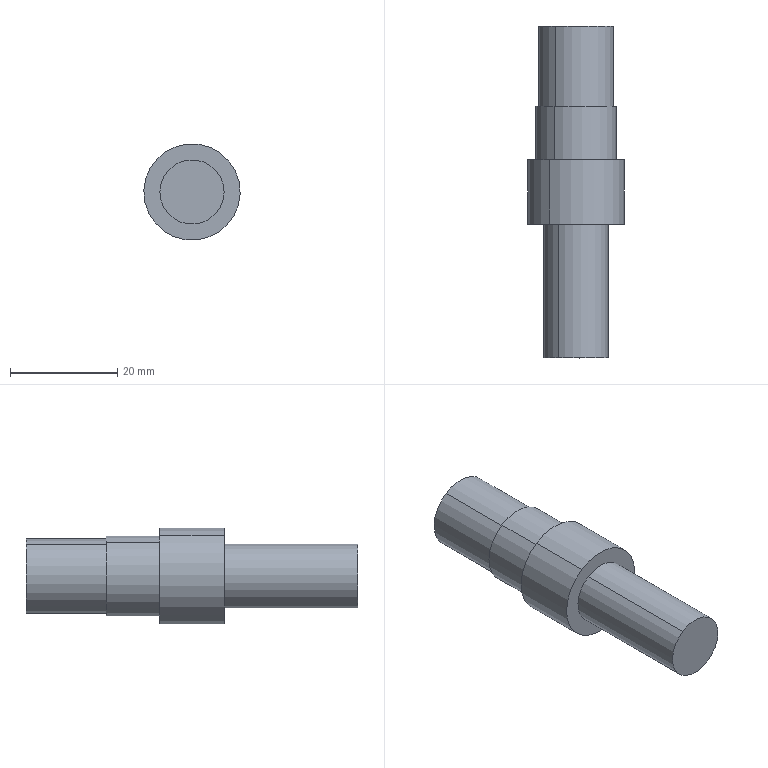Component | SolidWorks | CouplingAxis-1 | 1 solid | 13 faces | box 18 x 62 x 18 mm | volume 9957 mm3 | cylinder 8 | plane 5 | commonest cylinder face diameters 14 x2 15 x2 18 x2 12 x2
build123d program:
from build123d import *


with BuildPart() as part:
    # Sketch1 → Revolve1 (revolve)
    with BuildSketch(Plane.XY, mode=Mode.PRIVATE) as revolve1_sk:
        Polygon((0, 31.75), (6, 31.75), (6, 6.75), (9, 6.75), (9, -5.25), (7.5, -5.25), (7.5, -15.25), (7, -15.25), (7, -30.25), (0, -30.25), align=None)
    revolve(revolve1_sk.sketch.rotate(Axis((0, 0, 0), (0, 1, 0)), 90), axis=Axis((0, 0, 0), (0, 1, 0)))


solid = part.part

# Placed as in the assembly
solid = solid.moved(Location((-210.944, 520.733, 197.789), (180, 0, 0)))
STEP:
#1=COLOUR_RGB('',0.7922,0.8196,0.9333);
#2=FILL_AREA_STYLE_COLOUR('',#1);
#3=FILL_AREA_STYLE('',(#2));
#4=SURFACE_STYLE_FILL_AREA(#3);
#5=SURFACE_SIDE_STYLE('',(#4));
#6=SURFACE_STYLE_USAGE(.BOTH.,#5);
#7=PRESENTATION_STYLE_ASSIGNMENT((#6));
#8=CARTESIAN_POINT('',(-8.154,21.102,7.556));
#9=VERTEX_POINT('',#8);
#10=CARTESIAN_POINT('',(-8.456,21.102,8.018));
#11=VERTEX_POINT('',#10);
#12=CARTESIAN_POINT('',(-8.305,21.102,7.787));
#13=DIRECTION('',(0.,1.,0.));
#14=DIRECTION('',(0.5469,0.,-0.8372));
#15=AXIS2_PLACEMENT_3D('',#12,#13,#14);
#16=CIRCLE('',#15,0.2756);
#17=EDGE_CURVE('',#9,#11,#16,.T.);
#18=ORIENTED_EDGE('',*,*,#17,.T.);
#19=CARTESIAN_POINT('',(-8.456,21.692,8.018));
#20=VERTEX_POINT('',#19);
#21=CARTESIAN_POINT('',(-8.456,20.501,8.018));
#22=DIRECTION('',(0.,1.,0.));
#23=VECTOR('',#22,39.37);
#24=LINE('',#21,#23);
#25=EDGE_CURVE('',#11,#20,#24,.T.);
#26=ORIENTED_EDGE('',*,*,#25,.T.);
#27=CARTESIAN_POINT('',(-8.154,21.692,7.556));
#28=VERTEX_POINT('',#27);
#29=CARTESIAN_POINT('',(-8.305,21.692,7.787));
#30=DIRECTION('',(0.,1.,0.));
#31=DIRECTION('',(0.5469,0.,-0.8372));
#32=AXIS2_PLACEMENT_3D('',#29,#30,#31);
#33=CIRCLE('',#32,0.2756);
#34=EDGE_CURVE('',#28,#20,#33,.T.);
#35=ORIENTED_EDGE('',*,*,#34,.F.);
#36=CARTESIAN_POINT('',(-8.154,20.501,7.556));
#37=DIRECTION('',(0.,1.,0.));
#38=VECTOR('',#37,39.37);
#39=LINE('',#36,#38);
#40=EDGE_CURVE('',#9,#28,#39,.T.);
#41=ORIENTED_EDGE('',*,*,#40,.F.);
#42=EDGE_LOOP('',(#18,#26,#35,#41));
#43=FACE_OUTER_BOUND('',#42,.T.);
#44=CARTESIAN_POINT('',(-8.305,20.501,7.787));
#45=DIRECTION('',(0.,1.,0.));
#46=DIRECTION('',(0.5469,0.,-0.8372));
#47=AXIS2_PLACEMENT_3D('',#44,#45,#46);
#48=CYLINDRICAL_SURFACE('',#47,0.2756);
#49=ADVANCED_FACE('',(#43),#48,.T.);
#50=CARTESIAN_POINT('',(-8.143,20.708,7.54));
#51=VERTEX_POINT('',#50);
#52=CARTESIAN_POINT('',(-8.466,20.708,8.034));
#53=VERTEX_POINT('',#52);
#54=CARTESIAN_POINT('',(-8.305,20.708,7.787));
#55=DIRECTION('',(0.,1.,0.));
#56=DIRECTION('',(0.5469,0.,-0.8372));
#57=AXIS2_PLACEMENT_3D('',#54,#55,#56);
#58=CIRCLE('',#57,0.2953);
#59=EDGE_CURVE('',#51,#53,#58,.T.);
#60=ORIENTED_EDGE('',*,*,#59,.T.);
#61=CARTESIAN_POINT('',(-8.466,21.102,8.034));
#62=VERTEX_POINT('',#61);
#63=CARTESIAN_POINT('',(-8.466,20.501,8.034));
#64=DIRECTION('',(0.,1.,0.));
#65=VECTOR('',#64,39.37);
#66=LINE('',#63,#65);
#67=EDGE_CURVE('',#53,#62,#66,.T.);
#68=ORIENTED_EDGE('',*,*,#67,.T.);
#69=CARTESIAN_POINT('',(-8.143,21.102,7.54));
#70=VERTEX_POINT('',#69);
#71=CARTESIAN_POINT('',(-8.305,21.102,7.787));
#72=DIRECTION('',(0.,1.,0.));
#73=DIRECTION('',(0.5469,0.,-0.8372));
#74=AXIS2_PLACEMENT_3D('',#71,#72,#73);
#75=CIRCLE('',#74,0.2953);
#76=EDGE_CURVE('',#70,#62,#75,.T.);
#77=ORIENTED_EDGE('',*,*,#76,.F.);
#78=CARTESIAN_POINT('',(-8.143,20.501,7.54));
#79=DIRECTION('',(0.,1.,0.));
#80=VECTOR('',#79,39.37);
#81=LINE('',#78,#80);
#82=EDGE_CURVE('',#51,#70,#81,.T.);
#83=ORIENTED_EDGE('',*,*,#82,.F.);
#84=EDGE_LOOP('',(#60,#68,#77,#83));
#85=FACE_OUTER_BOUND('',#84,.T.);
#86=CARTESIAN_POINT('',(-8.305,20.501,7.787));
#87=DIRECTION('',(0.,1.,0.));
#88=DIRECTION('',(0.5469,0.,-0.8372));
#89=AXIS2_PLACEMENT_3D('',#86,#87,#88);
#90=CYLINDRICAL_SURFACE('',#89,0.2953);
#91=ADVANCED_FACE('',(#85),#90,.T.);
#92=CARTESIAN_POINT('',(-8.111,20.236,7.49));
#93=VERTEX_POINT('',#92);
#94=CARTESIAN_POINT('',(-8.499,20.236,8.084));
#95=VERTEX_POINT('',#94);
#96=CARTESIAN_POINT('',(-8.305,20.236,7.787));
#97=DIRECTION('',(0.,1.,0.));
#98=DIRECTION('',(0.5469,0.,-0.8372));
#99=AXIS2_PLACEMENT_3D('',#96,#97,#98);
#100=CIRCLE('',#99,0.3543);
#101=EDGE_CURVE('',#93,#95,#100,.T.);
#102=ORIENTED_EDGE('',*,*,#101,.T.);
#103=CARTESIAN_POINT('',(-8.499,20.708,8.084));
#104=VERTEX_POINT('',#103);
#105=CARTESIAN_POINT('',(-8.499,20.501,8.084));
#106=DIRECTION('',(0.,1.,0.));
#107=VECTOR('',#106,39.37);
#108=LINE('',#105,#107);
#109=EDGE_CURVE('',#95,#104,#108,.T.);
#110=ORIENTED_EDGE('',*,*,#109,.T.);
#111=CARTESIAN_POINT('',(-8.111,20.708,7.49));
#112=VERTEX_POINT('',#111);
#113=CARTESIAN_POINT('',(-8.305,20.708,7.787));
#114=DIRECTION('',(0.,1.,0.));
#115=DIRECTION('',(0.5469,0.,-0.8372));
#116=AXIS2_PLACEMENT_3D('',#113,#114,#115);
#117=CIRCLE('',#116,0.3543);
#118=EDGE_CURVE('',#112,#104,#117,.T.);
#119=ORIENTED_EDGE('',*,*,#118,.F.);
#120=CARTESIAN_POINT('',(-8.111,20.501,7.49));
#121=DIRECTION('',(0.,1.,0.));
#122=VECTOR('',#121,39.37);
#123=LINE('',#120,#122);
#124=EDGE_CURVE('',#93,#112,#123,.T.);
#125=ORIENTED_EDGE('',*,*,#124,.F.);
#126=EDGE_LOOP('',(#102,#110,#119,#125));
#127=FACE_OUTER_BOUND('',#126,.T.);
#128=CARTESIAN_POINT('',(-8.305,20.501,7.787));
#129=DIRECTION('',(0.,1.,0.));
#130=DIRECTION('',(0.5469,0.,-0.8372));
#131=AXIS2_PLACEMENT_3D('',#128,#129,#130);
#132=CYLINDRICAL_SURFACE('',#131,0.3543);
#133=ADVANCED_FACE('',(#127),#132,.T.);
#134=CARTESIAN_POINT('',(-8.176,19.251,7.589));
#135=VERTEX_POINT('',#134);
#136=CARTESIAN_POINT('',(-8.434,19.251,7.985));
#137=VERTEX_POINT('',#136);
#138=CARTESIAN_POINT('',(-8.305,19.251,7.787));
#139=DIRECTION('',(0.,1.,0.));
#140=DIRECTION('',(0.5469,0.,-0.8372));
#141=AXIS2_PLACEMENT_3D('',#138,#139,#140);
#142=CIRCLE('',#141,0.2362);
#143=EDGE_CURVE('',#135,#137,#142,.T.);
#144=ORIENTED_EDGE('',*,*,#143,.T.);
#145=CARTESIAN_POINT('',(-8.434,20.236,7.985));
#146=VERTEX_POINT('',#145);
#147=CARTESIAN_POINT('',(-8.434,20.501,7.985));
#148=DIRECTION('',(0.,1.,0.));
#149=VECTOR('',#148,39.37);
#150=LINE('',#147,#149);
#151=EDGE_CURVE('',#137,#146,#150,.T.);
#152=ORIENTED_EDGE('',*,*,#151,.T.);
#153=CARTESIAN_POINT('',(-8.176,20.236,7.589));
#154=VERTEX_POINT('',#153);
#155=CARTESIAN_POINT('',(-8.305,20.236,7.787));
#156=DIRECTION('',(0.,1.,0.));
#157=DIRECTION('',(0.5469,0.,-0.8372));
#158=AXIS2_PLACEMENT_3D('',#155,#156,#157);
#159=CIRCLE('',#158,0.2362);
#160=EDGE_CURVE('',#154,#146,#159,.T.);
#161=ORIENTED_EDGE('',*,*,#160,.F.);
#162=CARTESIAN_POINT('',(-8.176,20.501,7.589));
#163=DIRECTION('',(0.,1.,0.));
#164=VECTOR('',#163,39.37);
#165=LINE('',#162,#164);
#166=EDGE_CURVE('',#135,#154,#165,.T.);
#167=ORIENTED_EDGE('',*,*,#166,.F.);
#168=EDGE_LOOP('',(#144,#152,#161,#167));
#169=FACE_OUTER_BOUND('',#168,.T.);
#170=CARTESIAN_POINT('',(-8.305,20.501,7.787));
#171=DIRECTION('',(0.,1.,0.));
#172=DIRECTION('',(0.5469,0.,-0.8372));
#173=AXIS2_PLACEMENT_3D('',#170,#171,#172);
#174=CYLINDRICAL_SURFACE('',#173,0.2362);
#175=ADVANCED_FACE('',(#169),#174,.T.);
#176=ORIENTED_EDGE('',*,*,#143,.F.);
#177=CARTESIAN_POINT('',(-8.305,19.251,7.787));
#178=DIRECTION('',(0.,1.,0.));
#179=DIRECTION('',(0.5469,0.,-0.8372));
#180=AXIS2_PLACEMENT_3D('',#177,#178,#179);
#181=CIRCLE('',#180,0.2362);
#182=EDGE_CURVE('',#137,#135,#181,.T.);
#183=ORIENTED_EDGE('',*,*,#182,.F.);
#184=EDGE_LOOP('',(#176,#183));
#185=FACE_OUTER_BOUND('',#184,.T.);
#186=CARTESIAN_POINT('',(-8.305,19.251,7.787));
#187=DIRECTION('',(0.,-1.,0.));
#188=DIRECTION('',(-0.5469,0.,0.8372));
#189=AXIS2_PLACEMENT_3D('',#186,#187,#188);
#190=PLANE('',#189);
#191=ADVANCED_FACE('',(#185),#190,.T.);
#192=ORIENTED_EDGE('',*,*,#151,.F.);
#193=ORIENTED_EDGE('',*,*,#182,.T.);
#194=ORIENTED_EDGE('',*,*,#166,.T.);
#195=CARTESIAN_POINT('',(-8.305,20.236,7.787));
#196=DIRECTION('',(0.,1.,0.));
#197=DIRECTION('',(0.5469,0.,-0.8372));
#198=AXIS2_PLACEMENT_3D('',#195,#196,#197);
#199=CIRCLE('',#198,0.2362);
#200=EDGE_CURVE('',#146,#154,#199,.T.);
#201=ORIENTED_EDGE('',*,*,#200,.F.);
#202=EDGE_LOOP('',(#192,#193,#194,#201));
#203=FACE_OUTER_BOUND('',#202,.T.);
#204=CARTESIAN_POINT('',(-8.305,20.501,7.787));
#205=DIRECTION('',(0.,1.,0.));
#206=DIRECTION('',(0.5469,0.,-0.8372));
#207=AXIS2_PLACEMENT_3D('',#204,#205,#206);
#208=CYLINDRICAL_SURFACE('',#207,0.2362);
#209=ADVANCED_FACE('',(#203),#208,.T.);
#210=ORIENTED_EDGE('',*,*,#160,.T.);
#211=ORIENTED_EDGE('',*,*,#200,.T.);
#212=EDGE_LOOP('',(#210,#211));
#213=FACE_BOUND('',#212,.T.);
#214=ORIENTED_EDGE('',*,*,#101,.F.);
#215=CARTESIAN_POINT('',(-8.305,20.236,7.787));
#216=DIRECTION('',(0.,1.,0.));
#217=DIRECTION('',(0.5469,0.,-0.8372));
#218=AXIS2_PLACEMENT_3D('',#215,#216,#217);
#219=CIRCLE('',#218,0.3543);
#220=EDGE_CURVE('',#95,#93,#219,.T.);
#221=ORIENTED_EDGE('',*,*,#220,.F.);
#222=EDGE_LOOP('',(#214,#221));
#223=FACE_OUTER_BOUND('',#222,.T.);
#224=CARTESIAN_POINT('',(-8.503,20.236,7.658));
#225=DIRECTION('',(0.,-1.,0.));
#226=DIRECTION('',(-0.5469,0.,0.8372));
#227=AXIS2_PLACEMENT_3D('',#224,#225,#226);
#228=PLANE('',#227);
#229=ADVANCED_FACE('',(#213,#223),#228,.T.);
#230=ORIENTED_EDGE('',*,*,#109,.F.);
#231=ORIENTED_EDGE('',*,*,#220,.T.);
#232=ORIENTED_EDGE('',*,*,#124,.T.);
#233=CARTESIAN_POINT('',(-8.305,20.708,7.787));
#234=DIRECTION('',(0.,1.,0.));
#235=DIRECTION('',(0.5469,0.,-0.8372));
#236=AXIS2_PLACEMENT_3D('',#233,#234,#235);
#237=CIRCLE('',#236,0.3543);
#238=EDGE_CURVE('',#104,#112,#237,.T.);
#239=ORIENTED_EDGE('',*,*,#238,.F.);
#240=EDGE_LOOP('',(#230,#231,#232,#239));
#241=FACE_OUTER_BOUND('',#240,.T.);
#242=CARTESIAN_POINT('',(-8.305,20.501,7.787));
#243=DIRECTION('',(0.,1.,0.));
#244=DIRECTION('',(0.5469,0.,-0.8372));
#245=AXIS2_PLACEMENT_3D('',#242,#243,#244);
#246=CYLINDRICAL_SURFACE('',#245,0.3543);
#247=ADVANCED_FACE('',(#241),#246,.T.);
#248=ORIENTED_EDGE('',*,*,#118,.T.);
#249=ORIENTED_EDGE('',*,*,#238,.T.);
#250=EDGE_LOOP('',(#248,#249));
#251=FACE_OUTER_BOUND('',#250,.T.);
#252=ORIENTED_EDGE('',*,*,#59,.F.);
#253=CARTESIAN_POINT('',(-8.305,20.708,7.787));
#254=DIRECTION('',(0.,1.,0.));
#255=DIRECTION('',(0.5469,0.,-0.8372));
#256=AXIS2_PLACEMENT_3D('',#253,#254,#255);
#257=CIRCLE('',#256,0.2953);
#258=EDGE_CURVE('',#53,#51,#257,.T.);
#259=ORIENTED_EDGE('',*,*,#258,.F.);
#260=EDGE_LOOP('',(#252,#259));
#261=FACE_BOUND('',#260,.T.);
#262=CARTESIAN_POINT('',(-8.602,20.708,7.593));
#263=DIRECTION('',(0.,1.,0.));
#264=DIRECTION('',(0.5469,0.,-0.8372));
#265=AXIS2_PLACEMENT_3D('',#262,#263,#264);
#266=PLANE('',#265);
#267=ADVANCED_FACE('',(#251,#261),#266,.T.);
#268=ORIENTED_EDGE('',*,*,#67,.F.);
#269=ORIENTED_EDGE('',*,*,#258,.T.);
#270=ORIENTED_EDGE('',*,*,#82,.T.);
#271=CARTESIAN_POINT('',(-8.305,21.102,7.787));
#272=DIRECTION('',(0.,1.,0.));
#273=DIRECTION('',(0.5469,0.,-0.8372));
#274=AXIS2_PLACEMENT_3D('',#271,#272,#273);
#275=CIRCLE('',#274,0.2953);
#276=EDGE_CURVE('',#62,#70,#275,.T.);
#277=ORIENTED_EDGE('',*,*,#276,.F.);
#278=EDGE_LOOP('',(#268,#269,#270,#277));
#279=FACE_OUTER_BOUND('',#278,.T.);
#280=CARTESIAN_POINT('',(-8.305,20.501,7.787));
#281=DIRECTION('',(0.,1.,0.));
#282=DIRECTION('',(0.5469,0.,-0.8372));
#283=AXIS2_PLACEMENT_3D('',#280,#281,#282);
#284=CYLINDRICAL_SURFACE('',#283,0.2953);
#285=ADVANCED_FACE('',(#279),#284,.T.);
#286=ORIENTED_EDGE('',*,*,#76,.T.);
#287=ORIENTED_EDGE('',*,*,#276,.T.);
#288=EDGE_LOOP('',(#286,#287));
#289=FACE_OUTER_BOUND('',#288,.T.);
#290=ORIENTED_EDGE('',*,*,#17,.F.);
#291=CARTESIAN_POINT('',(-8.305,21.102,7.787));
#292=DIRECTION('',(0.,1.,0.));
#293=DIRECTION('',(0.5469,0.,-0.8372));
#294=AXIS2_PLACEMENT_3D('',#291,#292,#293);
#295=CIRCLE('',#294,0.2756);
#296=EDGE_CURVE('',#11,#9,#295,.T.);
#297=ORIENTED_EDGE('',*,*,#296,.F.);
#298=EDGE_LOOP('',(#290,#297));
#299=FACE_BOUND('',#298,.T.);
#300=CARTESIAN_POINT('',(-8.552,21.102,7.625));
#301=DIRECTION('',(0.,1.,0.));
#302=DIRECTION('',(0.5469,0.,-0.8372));
#303=AXIS2_PLACEMENT_3D('',#300,#301,#302);
#304=PLANE('',#303);
#305=ADVANCED_FACE('',(#289,#299),#304,.T.);
#306=ORIENTED_EDGE('',*,*,#25,.F.);
#307=ORIENTED_EDGE('',*,*,#296,.T.);
#308=ORIENTED_EDGE('',*,*,#40,.T.);
#309=CARTESIAN_POINT('',(-8.305,21.692,7.787));
#310=DIRECTION('',(0.,1.,0.));
#311=DIRECTION('',(0.5469,0.,-0.8372));
#312=AXIS2_PLACEMENT_3D('',#309,#310,#311);
#313=CIRCLE('',#312,0.2756);
#314=EDGE_CURVE('',#20,#28,#313,.T.);
#315=ORIENTED_EDGE('',*,*,#314,.F.);
#316=EDGE_LOOP('',(#306,#307,#308,#315));
#317=FACE_OUTER_BOUND('',#316,.T.);
#318=CARTESIAN_POINT('',(-8.305,20.501,7.787));
#319=DIRECTION('',(0.,1.,0.));
#320=DIRECTION('',(0.5469,0.,-0.8372));
#321=AXIS2_PLACEMENT_3D('',#318,#319,#320);
#322=CYLINDRICAL_SURFACE('',#321,0.2756);
#323=ADVANCED_FACE('',(#317),#322,.T.);
#324=ORIENTED_EDGE('',*,*,#34,.T.);
#325=ORIENTED_EDGE('',*,*,#314,.T.);
#326=EDGE_LOOP('',(#324,#325));
#327=FACE_OUTER_BOUND('',#326,.T.);
#328=CARTESIAN_POINT('',(-8.536,21.692,7.636));
#329=DIRECTION('',(0.,1.,0.));
#330=DIRECTION('',(0.5469,0.,-0.8372));
#331=AXIS2_PLACEMENT_3D('',#328,#329,#330);
#332=PLANE('',#331);
#333=ADVANCED_FACE('',(#327),#332,.T.);
#334=CLOSED_SHELL('',(#49,#91,#133,#175,#191,#209,#229,#247,#267,#285,#305,#323,#333));
#335=MANIFOLD_SOLID_BREP('',#334);
#336=STYLED_ITEM('',(#7),#335);
#337=(LENGTH_UNIT()NAMED_UNIT(*)SI_UNIT($,.METRE.));
#338=LENGTH_MEASURE_WITH_UNIT(LENGTH_MEASURE(0.0254),#337);
#339=DIMENSIONAL_EXPONENTS(1.,0.,0.,0.,0.,0.,0.);
#340=(CONVERSION_BASED_UNIT('',#338)LENGTH_UNIT()NAMED_UNIT(#339));
#341=UNCERTAINTY_MEASURE_WITH_UNIT(LENGTH_MEASURE(0.00001),#340,'','');
#342=(NAMED_UNIT(*)PLANE_ANGLE_UNIT()SI_UNIT($,.RADIAN.));
#343=(NAMED_UNIT(*)SI_UNIT($,.STERADIAN.)SOLID_ANGLE_UNIT());
#344=(GEOMETRIC_REPRESENTATION_CONTEXT(3)GLOBAL_UNCERTAINTY_ASSIGNED_CONTEXT((#341))GLOBAL_UNIT_ASSIGNED_CONTEXT((#340,#342,#343))REPRESENTATION_CONTEXT('',''));
#345=MECHANICAL_DESIGN_GEOMETRIC_PRESENTATION_REPRESENTATION('',(#336),#344);
#346=PRESENTATION_LAYER_ASSIGNMENT('','',(#336));
#347=CARTESIAN_POINT('',(0.,0.,0.));
#348=DIRECTION('',(0.,0.,1.));
#349=DIRECTION('',(1.,0.,0.));
#350=AXIS2_PLACEMENT_3D('',#347,#348,#349);
#351=(LENGTH_UNIT()NAMED_UNIT(*)SI_UNIT($,.METRE.));
#352=LENGTH_MEASURE_WITH_UNIT(LENGTH_MEASURE(0.0254),#351);
#353=DIMENSIONAL_EXPONENTS(1.,0.,0.,0.,0.,0.,0.);
#354=(CONVERSION_BASED_UNIT('',#352)LENGTH_UNIT()NAMED_UNIT(#353));
#355=UNCERTAINTY_MEASURE_WITH_UNIT(LENGTH_MEASURE(0.00001),#354,'','');
#356=(NAMED_UNIT(*)PLANE_ANGLE_UNIT()SI_UNIT($,.RADIAN.));
#357=(NAMED_UNIT(*)SI_UNIT($,.STERADIAN.)SOLID_ANGLE_UNIT());
#358=(GEOMETRIC_REPRESENTATION_CONTEXT(3)GLOBAL_UNCERTAINTY_ASSIGNED_CONTEXT((#355))GLOBAL_UNIT_ASSIGNED_CONTEXT((#354,#356,#357))REPRESENTATION_CONTEXT('',''));
#359=ADVANCED_BREP_SHAPE_REPRESENTATION('',(#335,#350),#358);